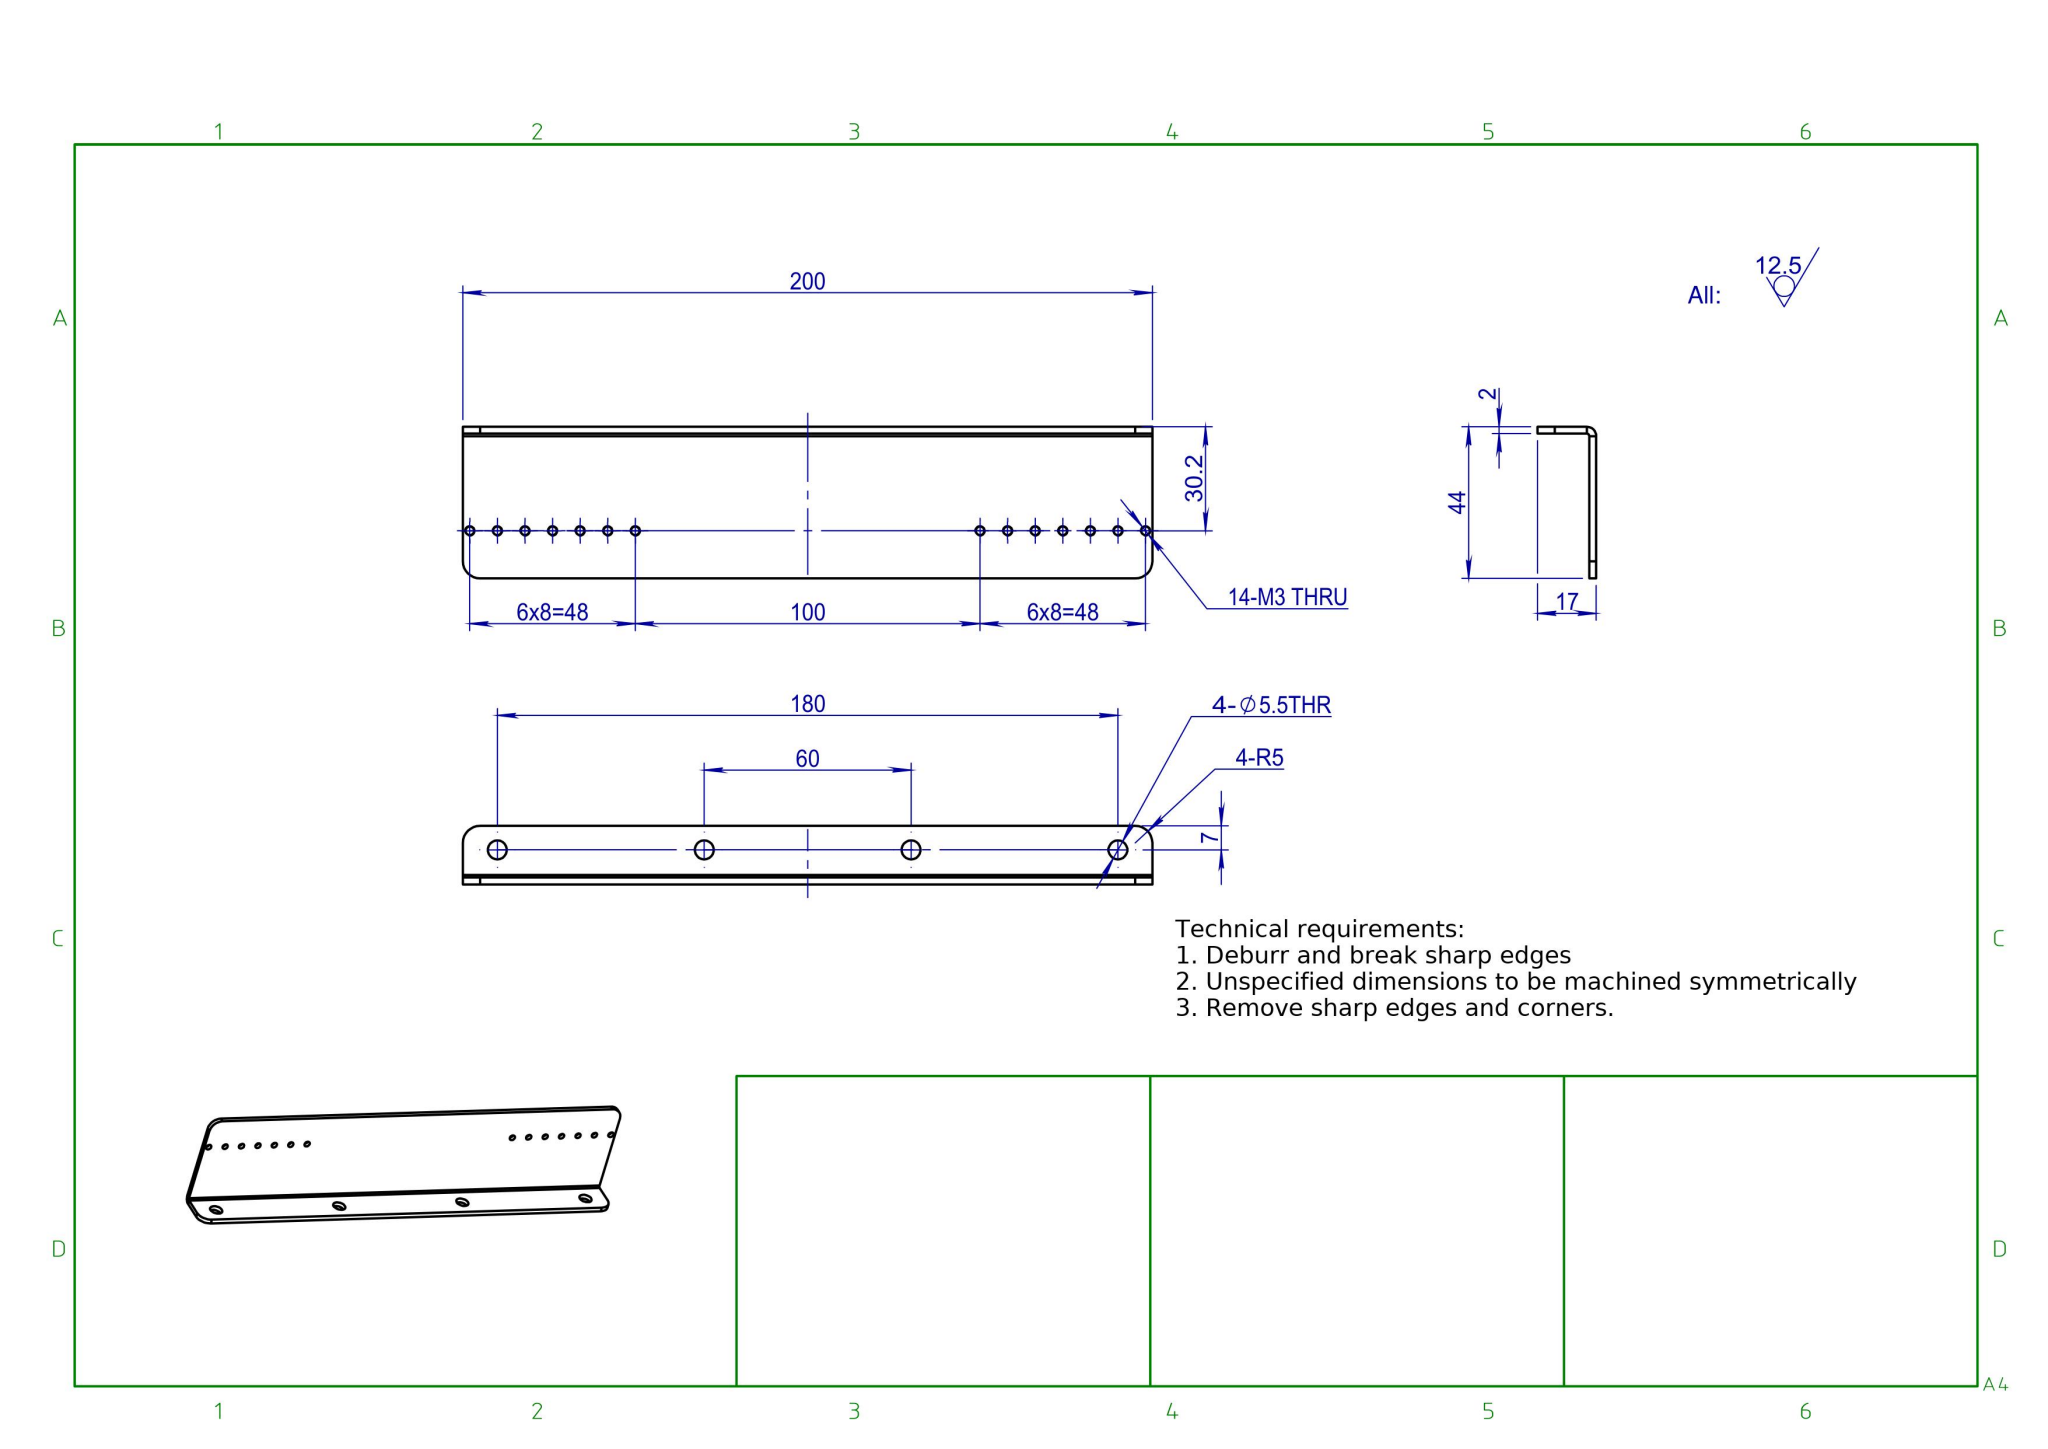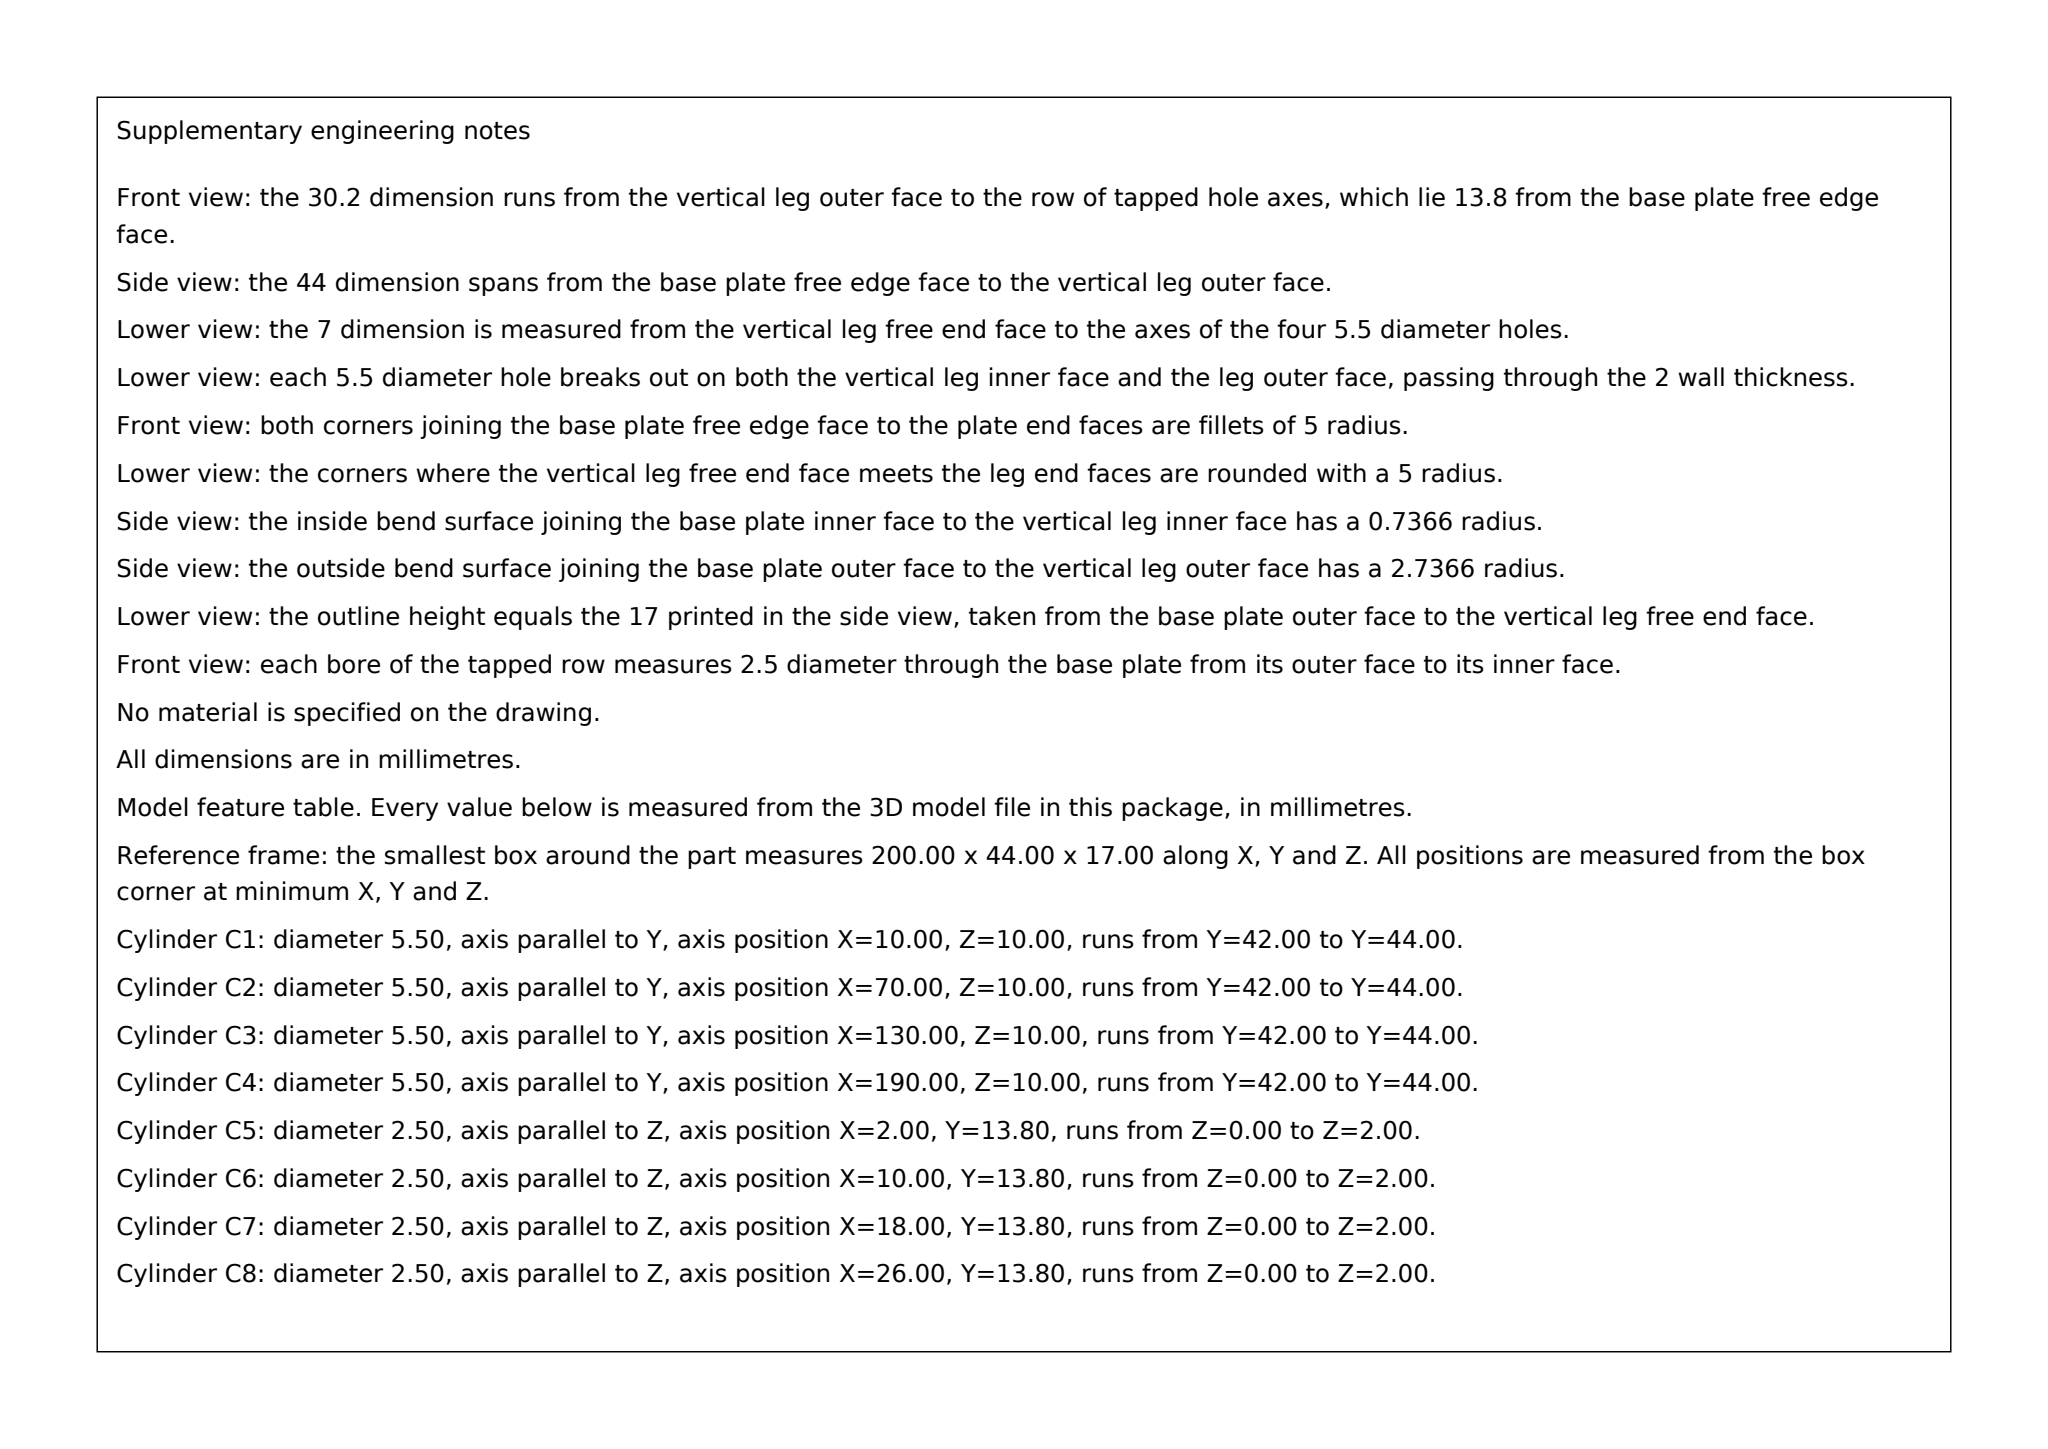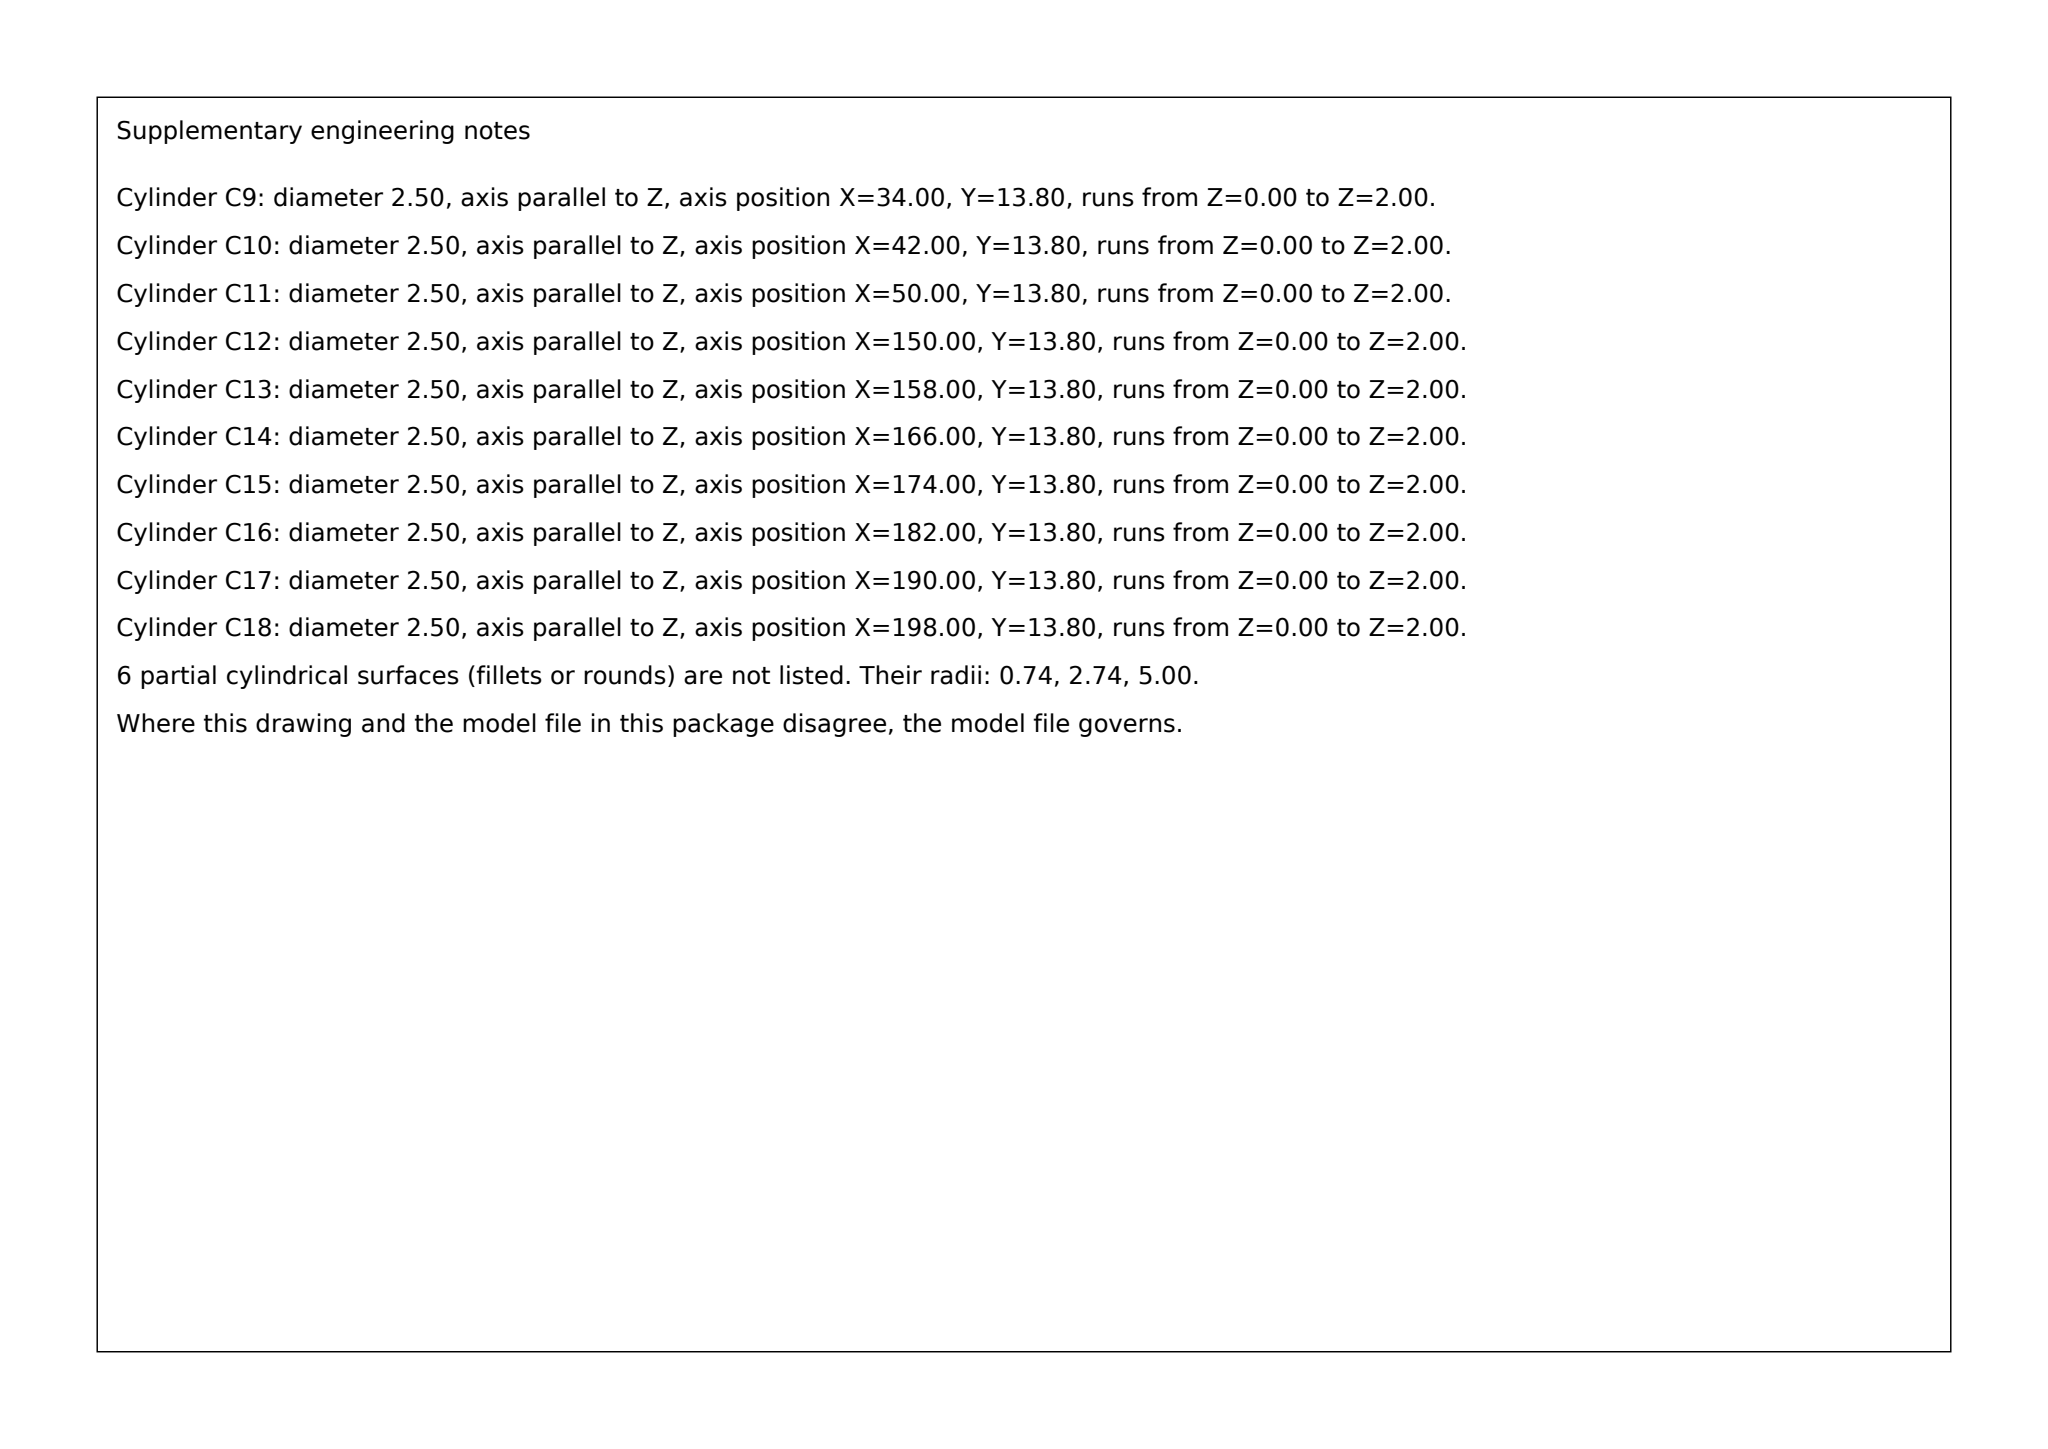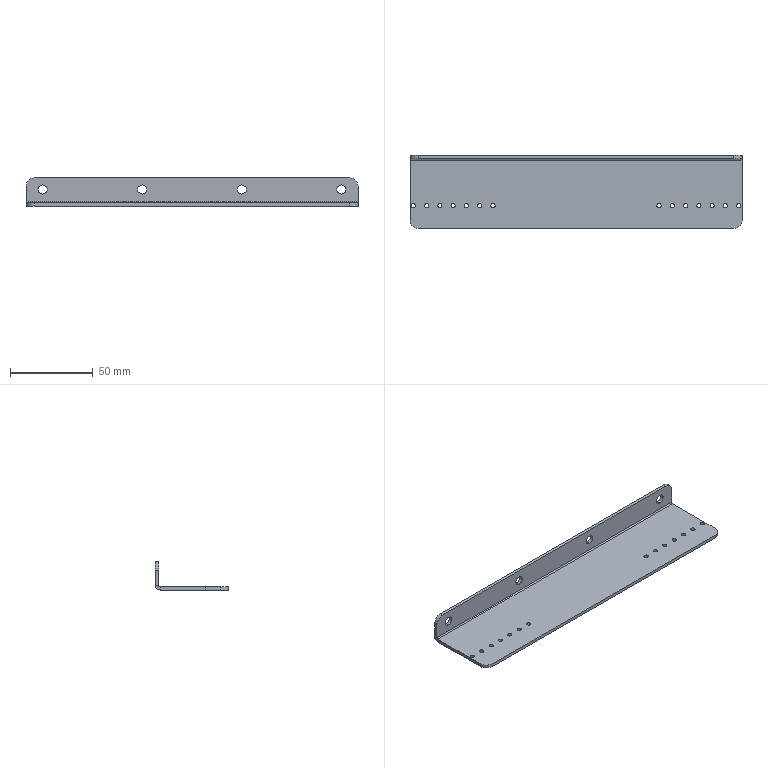Part | SolidWorks | mm | 1 solid | 54 faces | box 200 x 44 x 17 mm | volume 22931 mm3 | cylinder 42 | plane 12 | commonest cylinder face diameters 2.5 x28 5.5 x8 10 x4 5.473 x1 1.473 x1